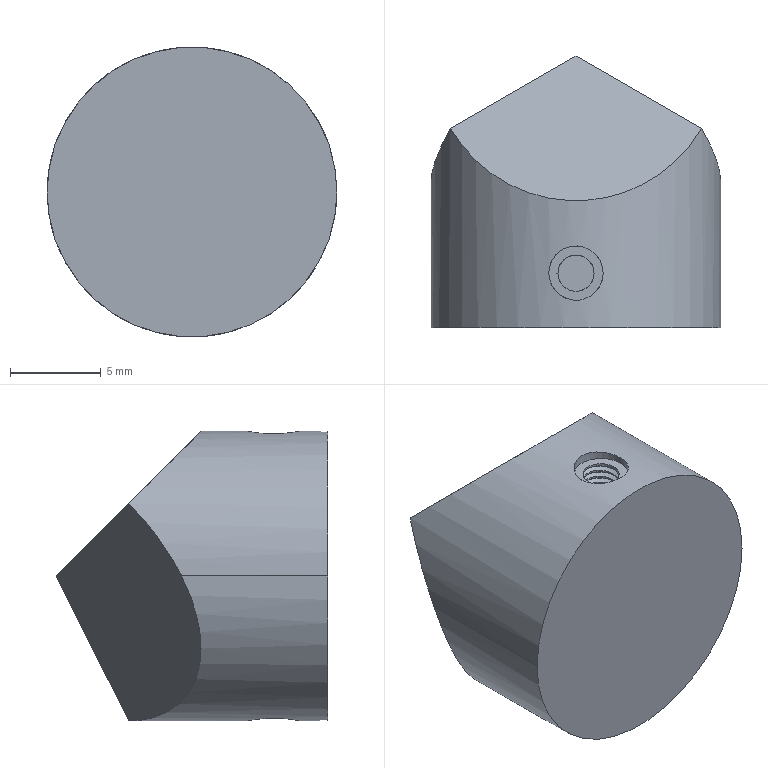Component | SolidWorks | CornerCubePrism-2 | 1 solid | 50 faces | volume 2107 mm3 | cylinder 32 | plane 12 | spline 6 | commonest cylinder face diameters 2 x26 3 x4 16 x2